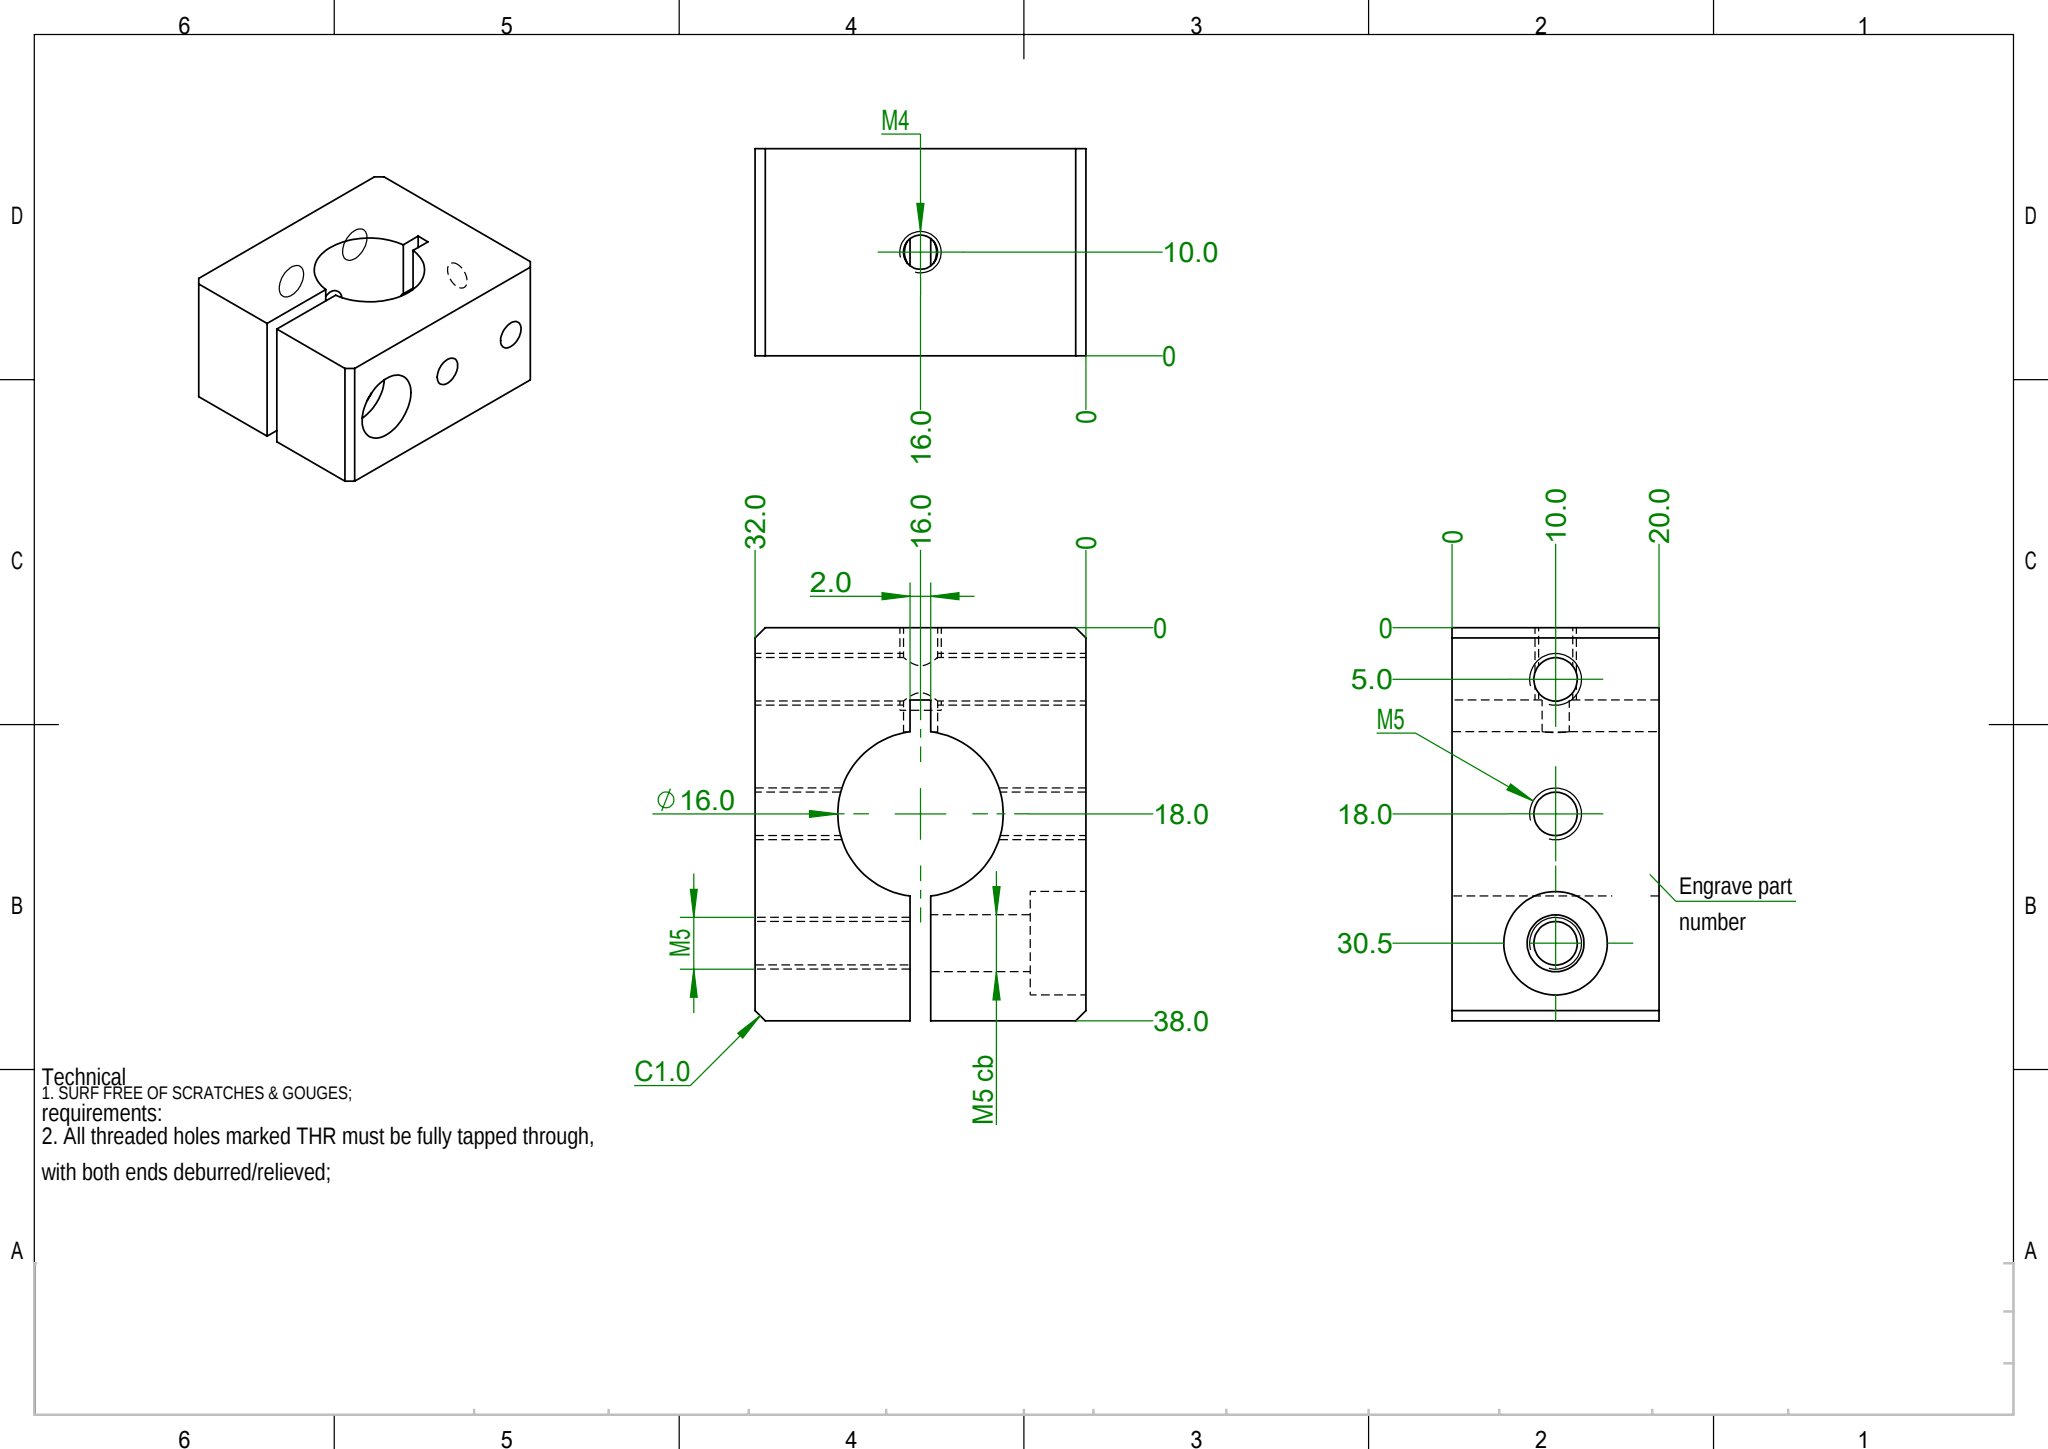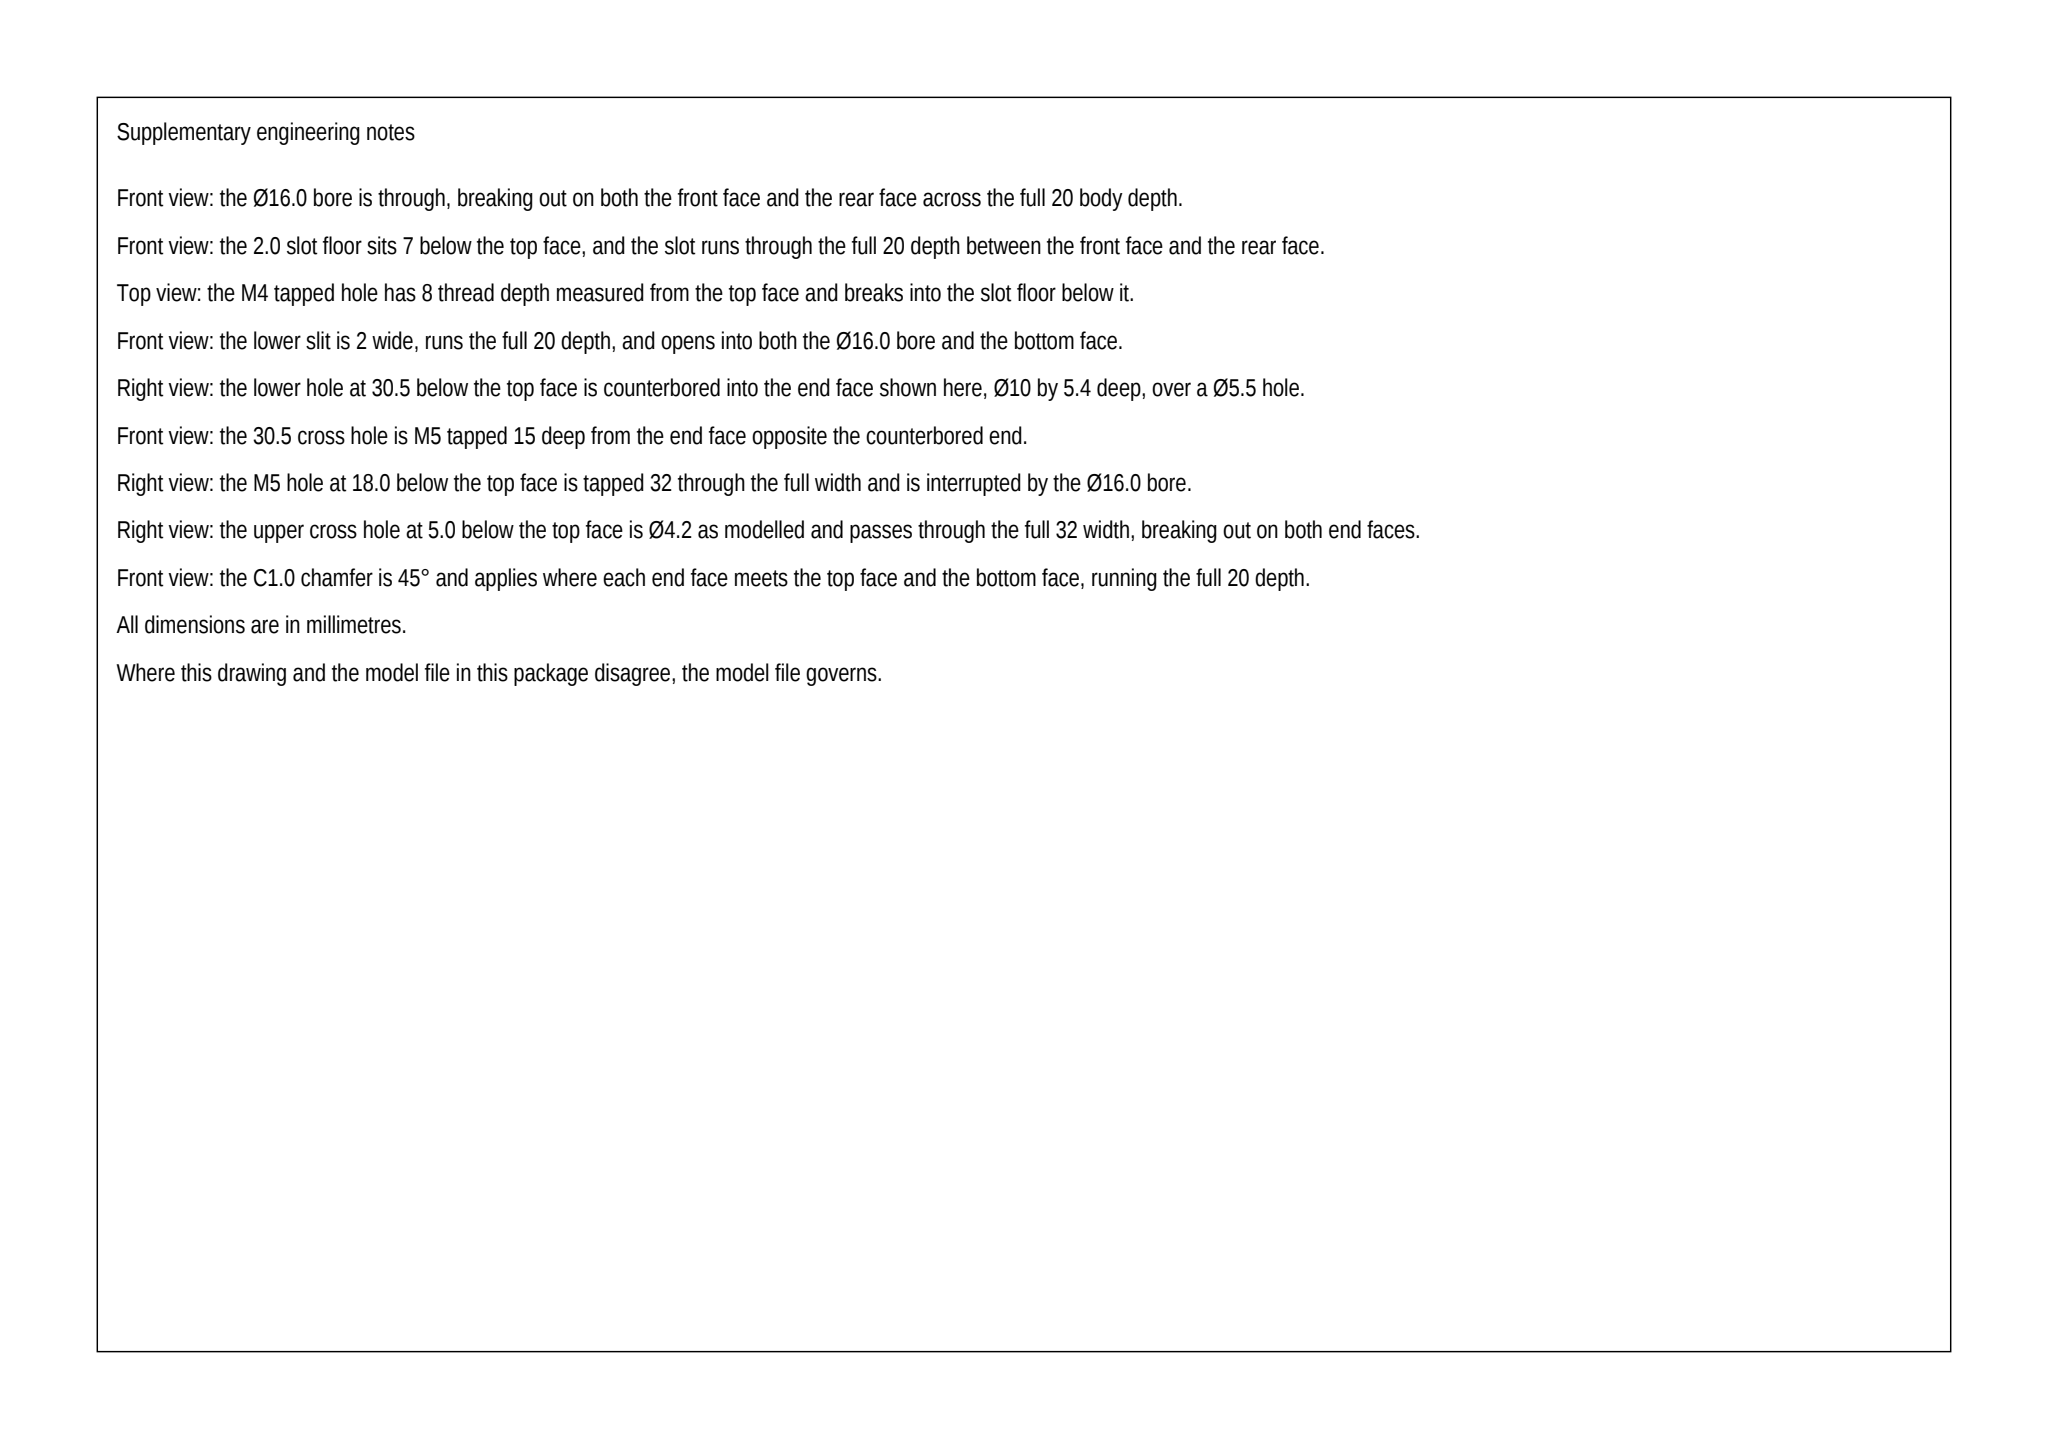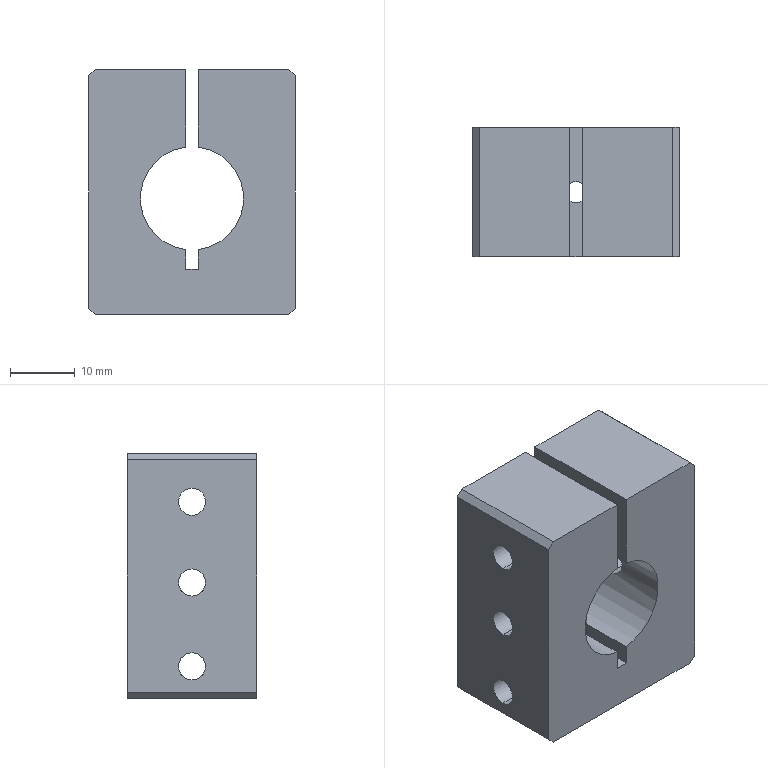Part | SolidWorks | mm | 1 solid | 41 faces | box 32 x 20 x 38 mm | volume 18096 mm3 | plane 20 | cylinder 18 | cone 3 | commonest cylinder face diameters 4.2 x8 3.3 x4 10 x2 5.5 x2 16 x2
Drawing notes:
SPLIT SLOT 2.0 WIDE THRU 20; CLOSED END 7.0 BELOW TOP FACE | from the solid: axis_planes x=15.0 & x=17.0 (2.0 gap) bounded by z=7.0 plane; slot open to z=38 and thru y=0-20
M4 DP 10.1; Ø3.3 TAP DRILL DP 11.1; NOT THRU | from the solid: Ø3.3 z-axis hole at (16,10): segments L=3.7 (z0-3.7) + L=3.8 (z6.3-10.1), 118° point on Ø3.3 adds 0.99
HOLE AT 5.0: M5 THR, Ø4.2 TAP DRILL, THRU 32 | from the solid: cyl Ø4.2 axis x at y=10,z=5.0, length 32.0 = full bbox width
M5 CB: Ø10 DP 5.4, THEN Ø5.5 DP 9.6 TO SLOT | from the solid: at y=10,z=30.5: Ø10 L=5.4 (x0-5.4), Ø5.5 L=9.6 (x5.4-15.0, slot face)
CLAMP HOLE 30.5: M5 THR DP 15 FAR SIDE; Ø5.5 CLR NEAR SIDE | from the solid: Ø4.2 axis x at y=10,z=30.5 L=15.0 (x17-32) tapped side; Ø5.5 L=9.6 + Ø10 cb L=5.4 on x=0 side